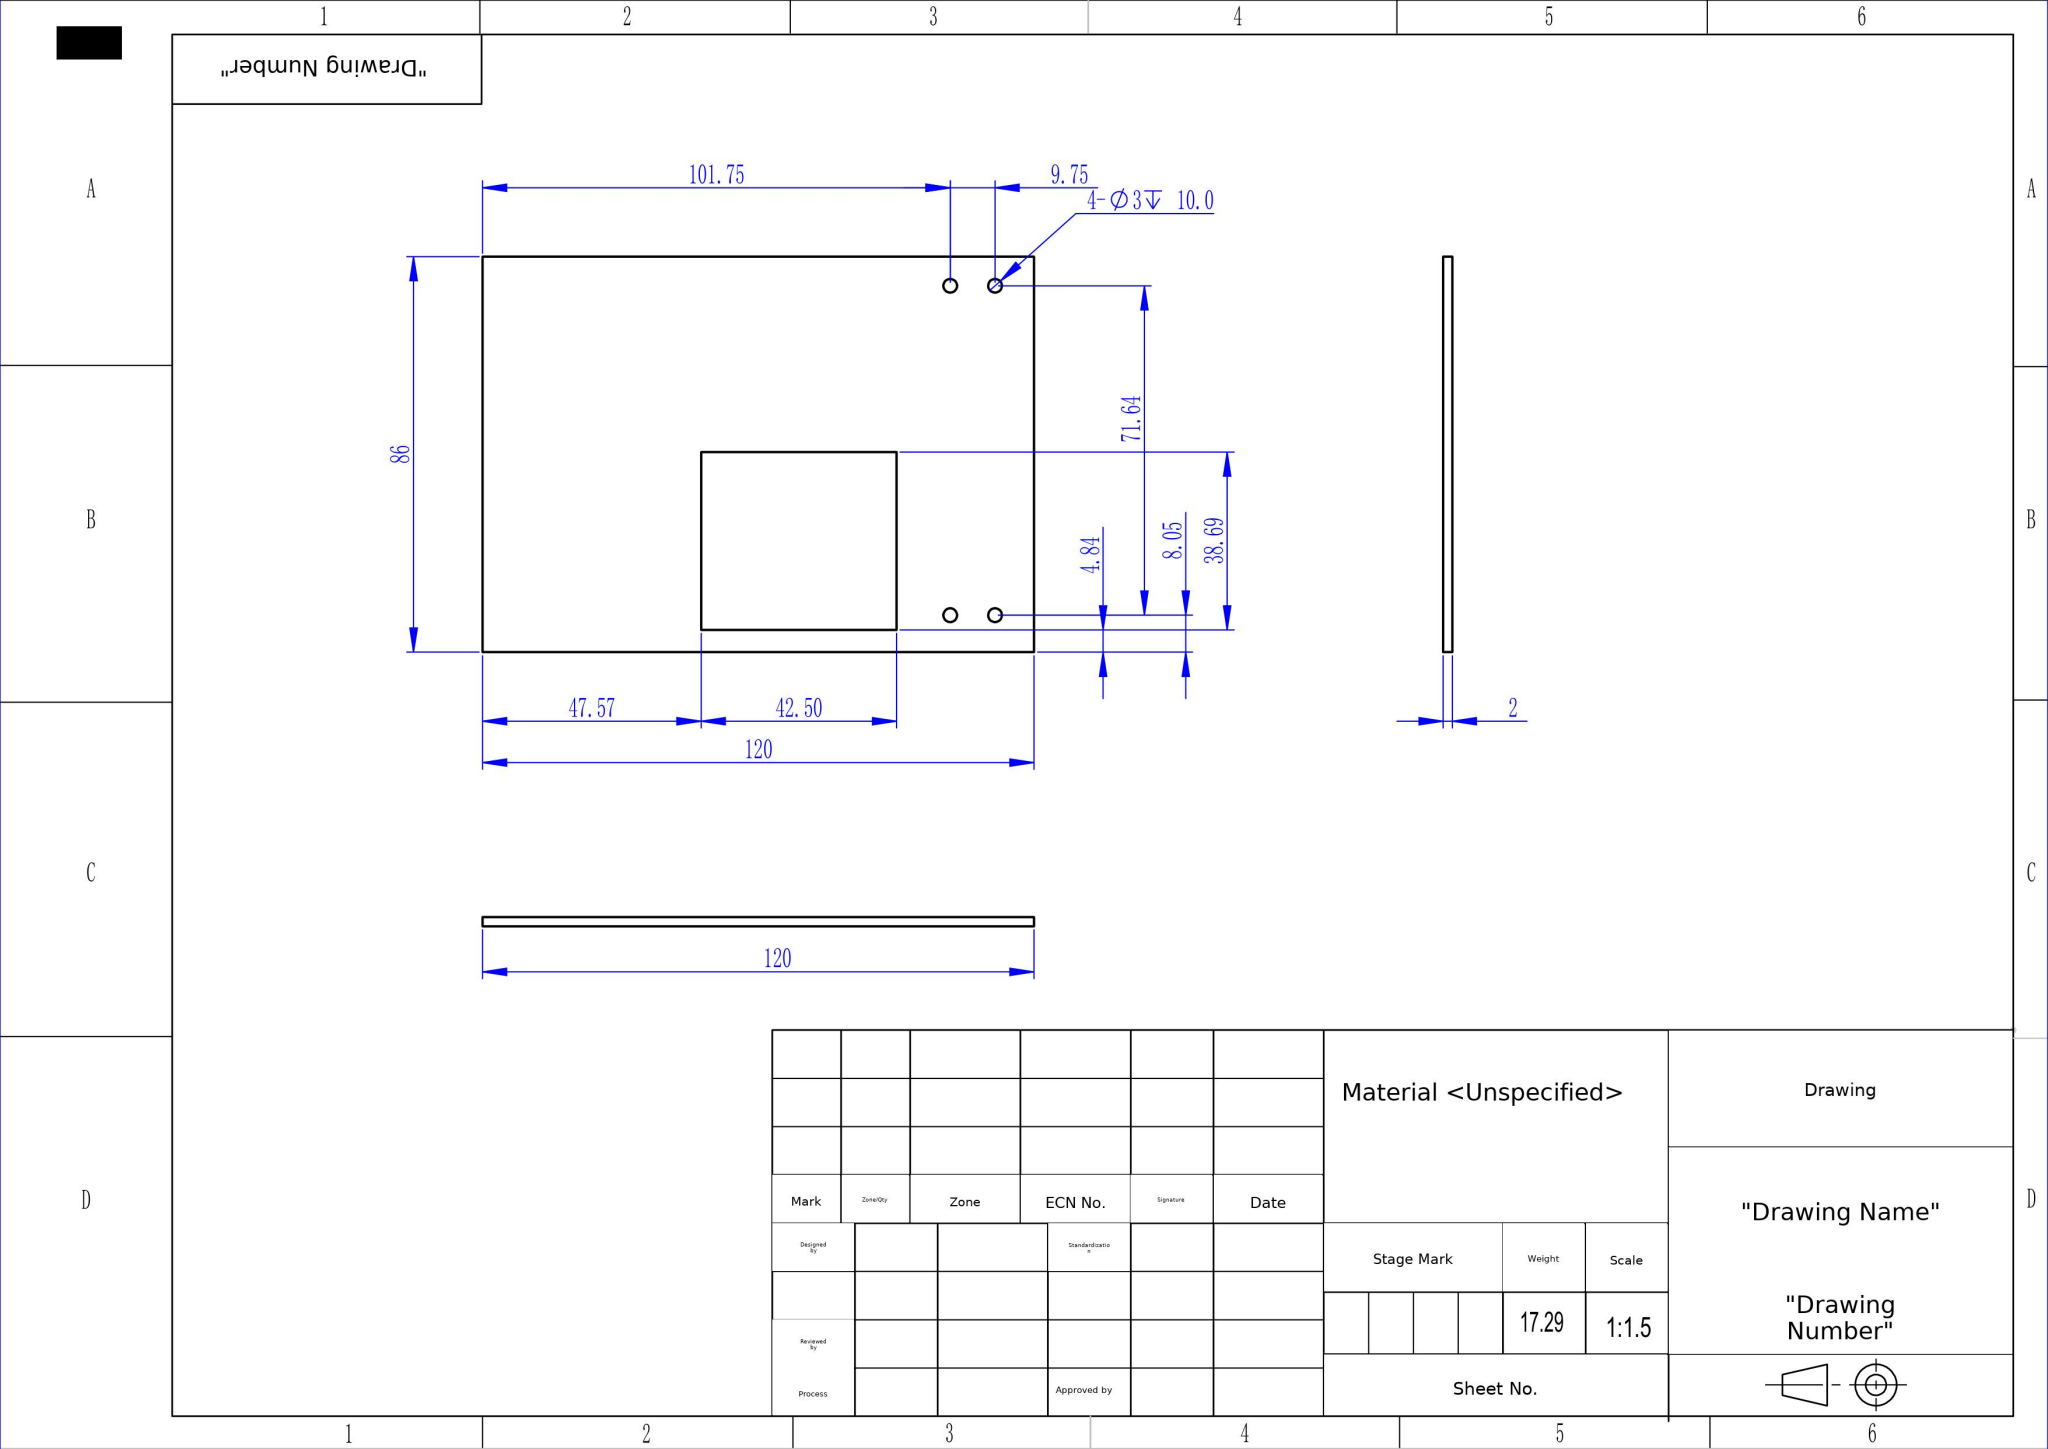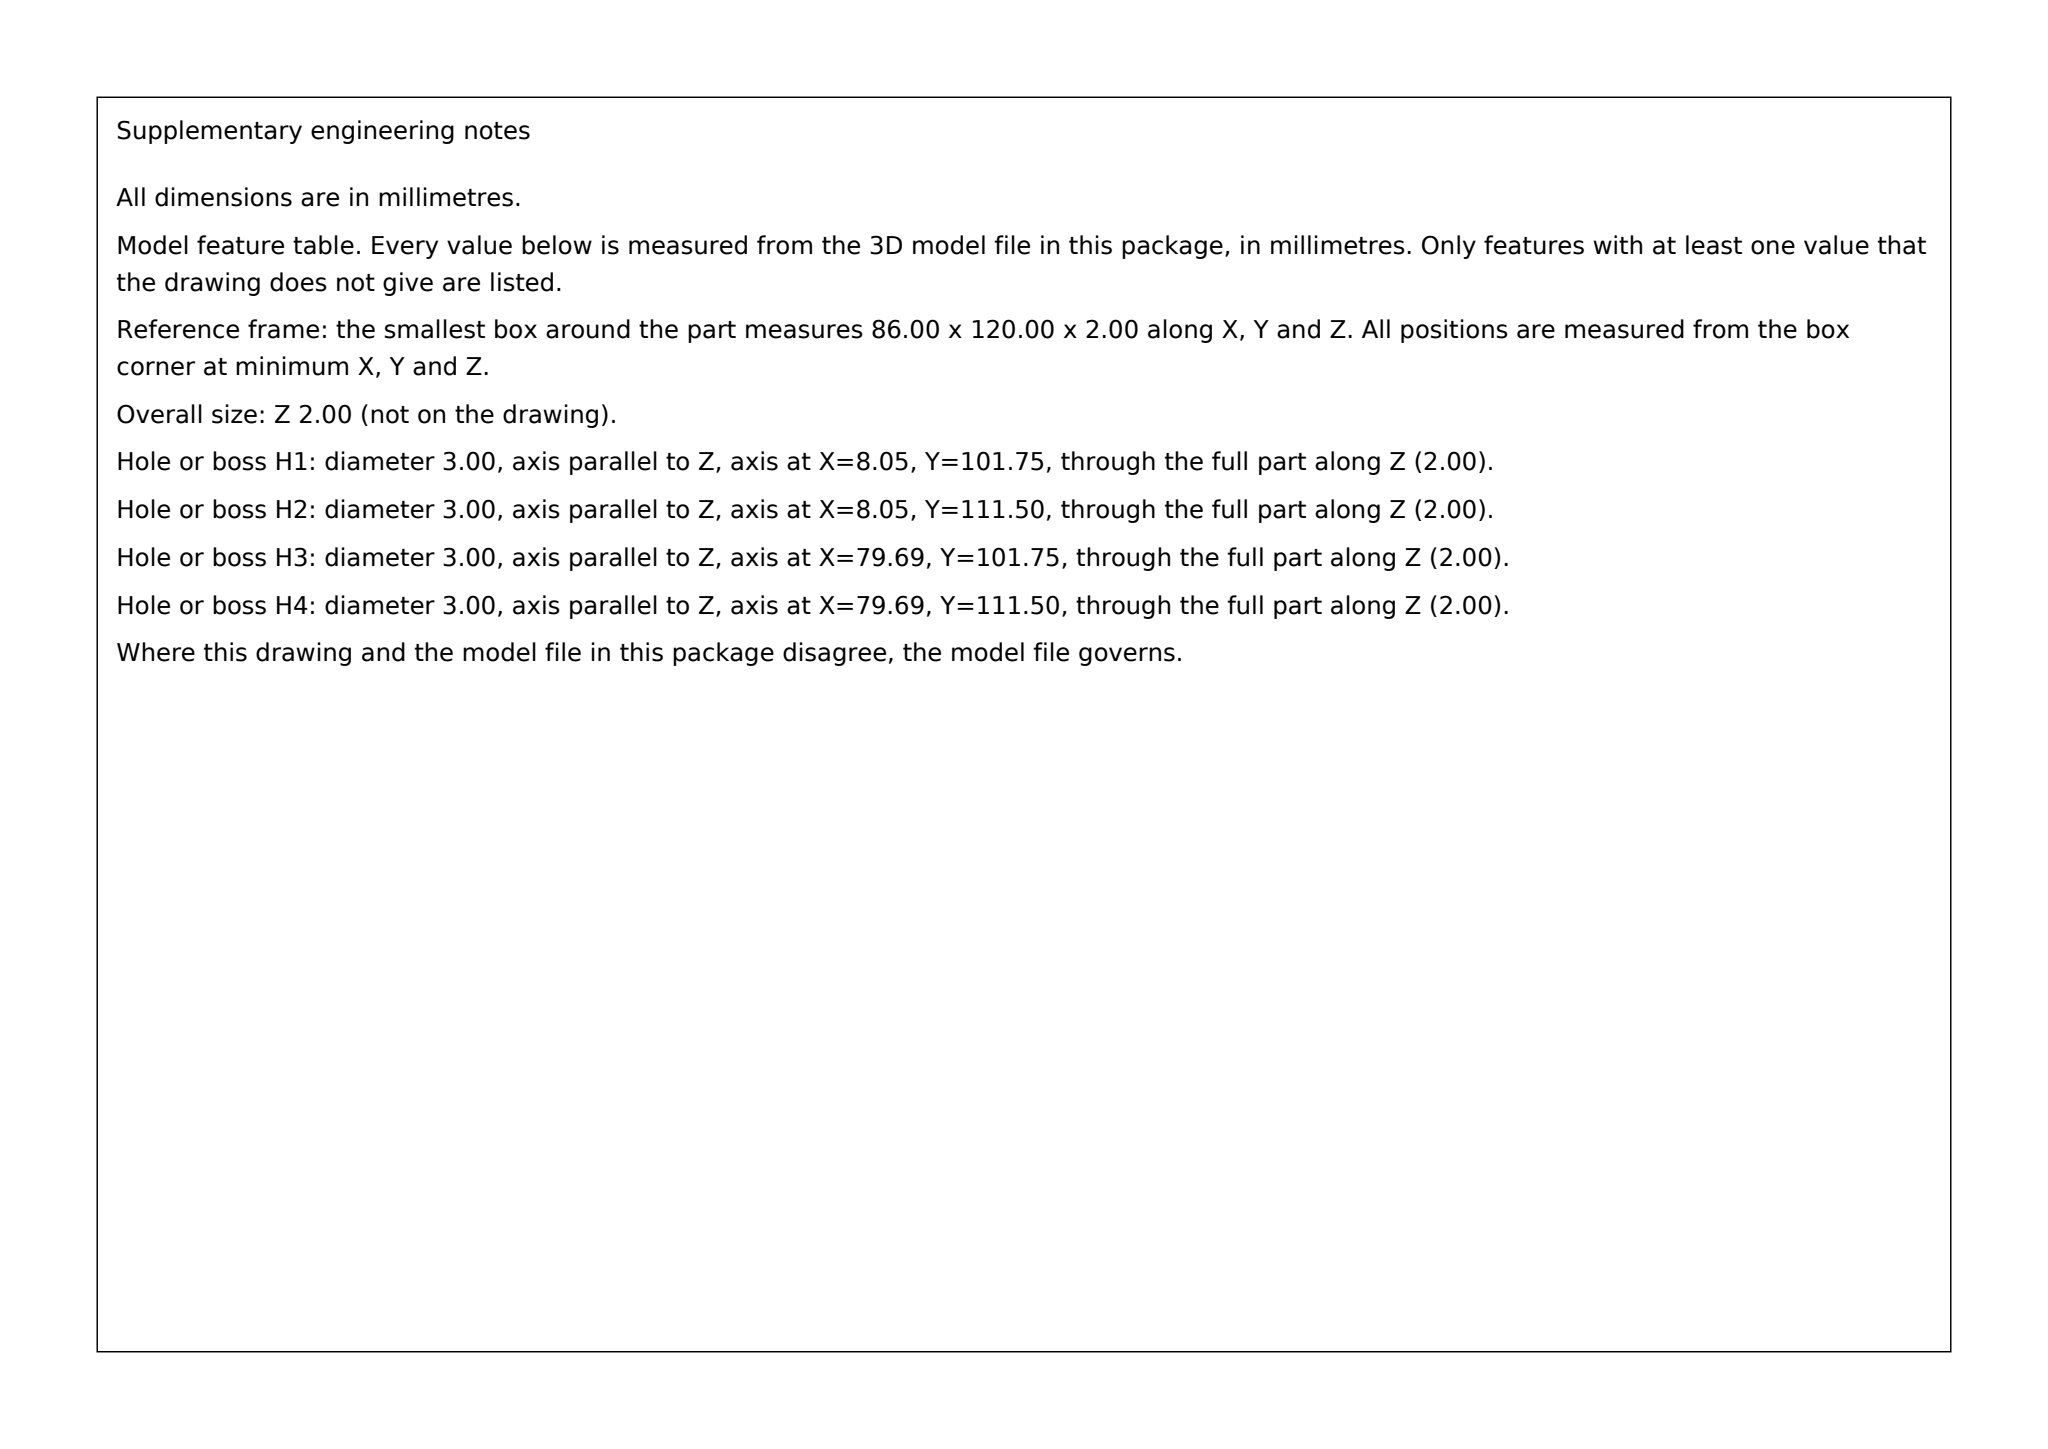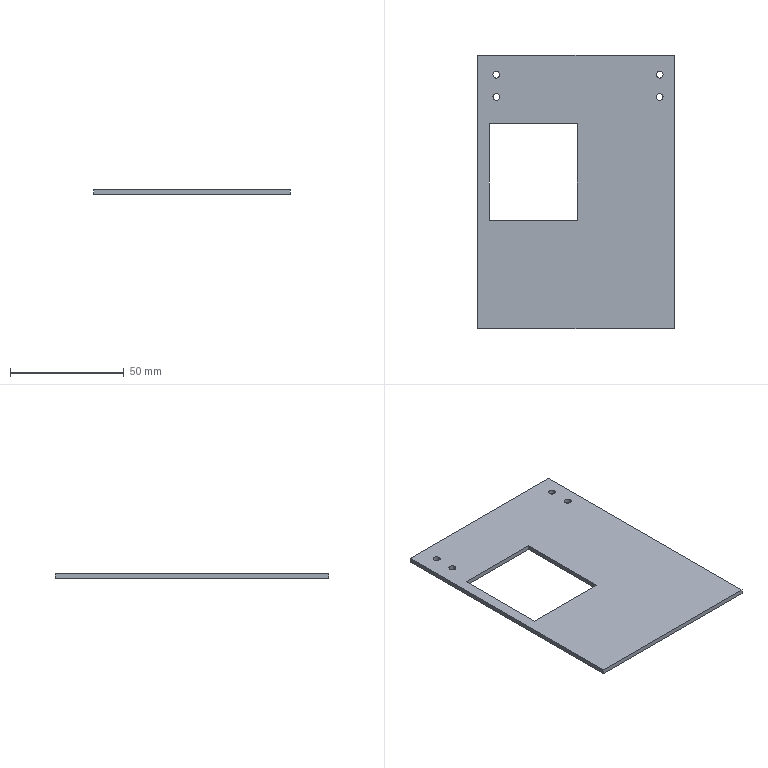Part | SolidWorks | mm | 1 solid | 18 faces | box 86 x 120 x 2 mm | volume 17294 mm3 | plane 10 | cylinder 8 | commonest cylinder face diameters 3 x8
build123d program:
from build123d import *

# Parameters (mm, degrees)
SKETCH1_W           = 86
SKETCH1_H           = 110
BOSS_EXTRUDE1_DEPTH = 2
SKETCH2_R           = 1.5
CUT_EXTRUDE1_DEPTH  = 10
SKETCH3_W           = 38.694
SKETCH3_H           = 42.503
CUT_EXTRUDE2_DEPTH  = 10
SKETCH4_W           = 86
SKETCH4_H           = 10
BOSS_EXTRUDE2_DEPTH = 2


with BuildPart() as part:
    # Sketch1 → Boss-Extrude1 (new body)
    with BuildSketch(Plane.XY):
        Rectangle(SKETCH1_W, SKETCH1_H)
    extrude(amount=BOSS_EXTRUDE1_DEPTH)

    # Sketch2 → Cut-Extrude1 (cut)
    with BuildSketch(Plane(origin=(0, 0, 0), x_dir=(-1, 0, 0), z_dir=(0, 0, -1))):
        with Locations((-36.686, 46.499)):
            Circle(SKETCH2_R)
        with Locations((34.95, 46.499)):
            Circle(SKETCH2_R)
        with Locations((-36.686, 36.747)):
            Circle(SKETCH2_R)
        with Locations((34.95, 36.747)):
            Circle(SKETCH2_R)
    extrude(amount=-CUT_EXTRUDE1_DEPTH, mode=Mode.SUBTRACT)

    # Sketch3 → Cut-Extrude2 (cut)
    with BuildSketch(Plane(origin=(0, 0, 0), x_dir=(-1, 0, 0), z_dir=(0, 0, -1))):
        with Locations((18.817, 3.817)):
            Rectangle(SKETCH3_W, SKETCH3_H)
    extrude(amount=-CUT_EXTRUDE2_DEPTH, mode=Mode.SUBTRACT)

    # Sketch4 → Boss-Extrude2 (add)
    with BuildSketch(Plane.XY.offset(2)):
        with Locations((0, -60)):
            Rectangle(SKETCH4_W, SKETCH4_H)
    extrude(amount=-BOSS_EXTRUDE2_DEPTH)


solid = part.part
STEP:
#1=CARTESIAN_POINT('',(-33.45,46.499,2.));
#2=VERTEX_POINT('',#1);
#3=CARTESIAN_POINT('',(-36.45,46.499,2.));
#4=VERTEX_POINT('',#3);
#5=CARTESIAN_POINT('',(-34.95,46.499,2.));
#6=DIRECTION('',(0.,0.,-1.));
#7=DIRECTION('',(-1.,0.,0.));
#8=AXIS2_PLACEMENT_3D('',#5,#6,#7);
#9=CIRCLE('',#8,1.5);
#10=EDGE_CURVE('',#2,#4,#9,.T.);
#11=ORIENTED_EDGE('',*,*,#10,.F.);
#12=CARTESIAN_POINT('',(-33.45,46.499,0.));
#13=VERTEX_POINT('',#12);
#14=CARTESIAN_POINT('',(-33.45,46.499,10.));
#15=DIRECTION('',(0.,0.,-1.));
#16=VECTOR('',#15,1000.);
#17=LINE('',#14,#16);
#18=EDGE_CURVE('',#2,#13,#17,.T.);
#19=ORIENTED_EDGE('',*,*,#18,.T.);
#20=CARTESIAN_POINT('',(-36.45,46.499,0.));
#21=VERTEX_POINT('',#20);
#22=CARTESIAN_POINT('',(-34.95,46.499,0.));
#23=DIRECTION('',(0.,0.,-1.));
#24=DIRECTION('',(-1.,0.,0.));
#25=AXIS2_PLACEMENT_3D('',#22,#23,#24);
#26=CIRCLE('',#25,1.5);
#27=EDGE_CURVE('',#13,#21,#26,.T.);
#28=ORIENTED_EDGE('',*,*,#27,.T.);
#29=CARTESIAN_POINT('',(-36.45,46.499,10.));
#30=DIRECTION('',(0.,0.,-1.));
#31=VECTOR('',#30,1000.);
#32=LINE('',#29,#31);
#33=EDGE_CURVE('',#4,#21,#32,.T.);
#34=ORIENTED_EDGE('',*,*,#33,.F.);
#35=EDGE_LOOP('',(#11,#19,#28,#34));
#36=FACE_OUTER_BOUND('',#35,.T.);
#37=CARTESIAN_POINT('',(-34.95,46.499,10.));
#38=DIRECTION('',(0.,0.,-1.));
#39=DIRECTION('',(-1.,0.,0.));
#40=AXIS2_PLACEMENT_3D('',#37,#38,#39);
#41=CYLINDRICAL_SURFACE('',#40,1.5);
#42=ADVANCED_FACE('',(#36),#41,.F.);
#43=CARTESIAN_POINT('',(38.186,36.747,2.));
#44=VERTEX_POINT('',#43);
#45=CARTESIAN_POINT('',(35.186,36.747,2.));
#46=VERTEX_POINT('',#45);
#47=CARTESIAN_POINT('',(36.686,36.747,2.));
#48=DIRECTION('',(0.,0.,-1.));
#49=DIRECTION('',(-1.,0.,0.));
#50=AXIS2_PLACEMENT_3D('',#47,#48,#49);
#51=CIRCLE('',#50,1.5);
#52=EDGE_CURVE('',#44,#46,#51,.T.);
#53=ORIENTED_EDGE('',*,*,#52,.F.);
#54=CARTESIAN_POINT('',(38.186,36.747,0.));
#55=VERTEX_POINT('',#54);
#56=CARTESIAN_POINT('',(38.186,36.747,10.));
#57=DIRECTION('',(0.,0.,-1.));
#58=VECTOR('',#57,1000.);
#59=LINE('',#56,#58);
#60=EDGE_CURVE('',#44,#55,#59,.T.);
#61=ORIENTED_EDGE('',*,*,#60,.T.);
#62=CARTESIAN_POINT('',(35.186,36.747,0.));
#63=VERTEX_POINT('',#62);
#64=CARTESIAN_POINT('',(36.686,36.747,0.));
#65=DIRECTION('',(0.,0.,-1.));
#66=DIRECTION('',(-1.,0.,0.));
#67=AXIS2_PLACEMENT_3D('',#64,#65,#66);
#68=CIRCLE('',#67,1.5);
#69=EDGE_CURVE('',#55,#63,#68,.T.);
#70=ORIENTED_EDGE('',*,*,#69,.T.);
#71=CARTESIAN_POINT('',(35.186,36.747,10.));
#72=DIRECTION('',(0.,0.,-1.));
#73=VECTOR('',#72,1000.);
#74=LINE('',#71,#73);
#75=EDGE_CURVE('',#46,#63,#74,.T.);
#76=ORIENTED_EDGE('',*,*,#75,.F.);
#77=EDGE_LOOP('',(#53,#61,#70,#76));
#78=FACE_OUTER_BOUND('',#77,.T.);
#79=CARTESIAN_POINT('',(36.686,36.747,10.));
#80=DIRECTION('',(0.,0.,-1.));
#81=DIRECTION('',(-1.,0.,0.));
#82=AXIS2_PLACEMENT_3D('',#79,#80,#81);
#83=CYLINDRICAL_SURFACE('',#82,1.5);
#84=ADVANCED_FACE('',(#78),#83,.F.);
#85=CARTESIAN_POINT('',(-33.45,36.747,2.));
#86=VERTEX_POINT('',#85);
#87=CARTESIAN_POINT('',(-36.45,36.747,2.));
#88=VERTEX_POINT('',#87);
#89=CARTESIAN_POINT('',(-34.95,36.747,2.));
#90=DIRECTION('',(0.,0.,-1.));
#91=DIRECTION('',(-1.,0.,0.));
#92=AXIS2_PLACEMENT_3D('',#89,#90,#91);
#93=CIRCLE('',#92,1.5);
#94=EDGE_CURVE('',#86,#88,#93,.T.);
#95=ORIENTED_EDGE('',*,*,#94,.F.);
#96=CARTESIAN_POINT('',(-33.45,36.747,0.));
#97=VERTEX_POINT('',#96);
#98=CARTESIAN_POINT('',(-33.45,36.747,10.));
#99=DIRECTION('',(0.,0.,-1.));
#100=VECTOR('',#99,1000.);
#101=LINE('',#98,#100);
#102=EDGE_CURVE('',#86,#97,#101,.T.);
#103=ORIENTED_EDGE('',*,*,#102,.T.);
#104=CARTESIAN_POINT('',(-36.45,36.747,0.));
#105=VERTEX_POINT('',#104);
#106=CARTESIAN_POINT('',(-34.95,36.747,0.));
#107=DIRECTION('',(0.,0.,-1.));
#108=DIRECTION('',(-1.,0.,0.));
#109=AXIS2_PLACEMENT_3D('',#106,#107,#108);
#110=CIRCLE('',#109,1.5);
#111=EDGE_CURVE('',#97,#105,#110,.T.);
#112=ORIENTED_EDGE('',*,*,#111,.T.);
#113=CARTESIAN_POINT('',(-36.45,36.747,10.));
#114=DIRECTION('',(0.,0.,-1.));
#115=VECTOR('',#114,1000.);
#116=LINE('',#113,#115);
#117=EDGE_CURVE('',#88,#105,#116,.T.);
#118=ORIENTED_EDGE('',*,*,#117,.F.);
#119=EDGE_LOOP('',(#95,#103,#112,#118));
#120=FACE_OUTER_BOUND('',#119,.T.);
#121=CARTESIAN_POINT('',(-34.95,36.747,10.));
#122=DIRECTION('',(0.,0.,-1.));
#123=DIRECTION('',(-1.,0.,0.));
#124=AXIS2_PLACEMENT_3D('',#121,#122,#123);
#125=CYLINDRICAL_SURFACE('',#124,1.5);
#126=ADVANCED_FACE('',(#120),#125,.F.);
#127=CARTESIAN_POINT('',(38.186,46.499,2.));
#128=VERTEX_POINT('',#127);
#129=CARTESIAN_POINT('',(35.186,46.499,2.));
#130=VERTEX_POINT('',#129);
#131=CARTESIAN_POINT('',(36.686,46.499,2.));
#132=DIRECTION('',(0.,0.,-1.));
#133=DIRECTION('',(-1.,0.,0.));
#134=AXIS2_PLACEMENT_3D('',#131,#132,#133);
#135=CIRCLE('',#134,1.5);
#136=EDGE_CURVE('',#128,#130,#135,.T.);
#137=ORIENTED_EDGE('',*,*,#136,.F.);
#138=CARTESIAN_POINT('',(38.186,46.499,0.));
#139=VERTEX_POINT('',#138);
#140=CARTESIAN_POINT('',(38.186,46.499,10.));
#141=DIRECTION('',(0.,0.,-1.));
#142=VECTOR('',#141,1000.);
#143=LINE('',#140,#142);
#144=EDGE_CURVE('',#128,#139,#143,.T.);
#145=ORIENTED_EDGE('',*,*,#144,.T.);
#146=CARTESIAN_POINT('',(35.186,46.499,0.));
#147=VERTEX_POINT('',#146);
#148=CARTESIAN_POINT('',(36.686,46.499,0.));
#149=DIRECTION('',(0.,0.,-1.));
#150=DIRECTION('',(-1.,0.,0.));
#151=AXIS2_PLACEMENT_3D('',#148,#149,#150);
#152=CIRCLE('',#151,1.5);
#153=EDGE_CURVE('',#139,#147,#152,.T.);
#154=ORIENTED_EDGE('',*,*,#153,.T.);
#155=CARTESIAN_POINT('',(35.186,46.499,10.));
#156=DIRECTION('',(0.,0.,-1.));
#157=VECTOR('',#156,1000.);
#158=LINE('',#155,#157);
#159=EDGE_CURVE('',#130,#147,#158,.T.);
#160=ORIENTED_EDGE('',*,*,#159,.F.);
#161=EDGE_LOOP('',(#137,#145,#154,#160));
#162=FACE_OUTER_BOUND('',#161,.T.);
#163=CARTESIAN_POINT('',(36.686,46.499,10.));
#164=DIRECTION('',(0.,0.,-1.));
#165=DIRECTION('',(-1.,0.,0.));
#166=AXIS2_PLACEMENT_3D('',#163,#164,#165);
#167=CYLINDRICAL_SURFACE('',#166,1.5);
#168=ADVANCED_FACE('',(#162),#167,.F.);
#169=CARTESIAN_POINT('',(43.,-65.,0.));
#170=VERTEX_POINT('',#169);
#171=CARTESIAN_POINT('',(43.,55.,0.));
#172=VERTEX_POINT('',#171);
#173=CARTESIAN_POINT('',(43.,-55.,0.));
#174=DIRECTION('',(0.,1.,0.));
#175=VECTOR('',#174,1000.);
#176=LINE('',#173,#175);
#177=EDGE_CURVE('',#170,#172,#176,.T.);
#178=ORIENTED_EDGE('',*,*,#177,.T.);
#179=CARTESIAN_POINT('',(43.,55.,2.));
#180=VERTEX_POINT('',#179);
#181=CARTESIAN_POINT('',(43.,55.,2.));
#182=DIRECTION('',(0.,0.,-1.));
#183=VECTOR('',#182,1000.);
#184=LINE('',#181,#183);
#185=EDGE_CURVE('',#180,#172,#184,.T.);
#186=ORIENTED_EDGE('',*,*,#185,.F.);
#187=CARTESIAN_POINT('',(43.,-65.,2.));
#188=VERTEX_POINT('',#187);
#189=CARTESIAN_POINT('',(43.,-55.,2.));
#190=DIRECTION('',(0.,1.,0.));
#191=VECTOR('',#190,1000.);
#192=LINE('',#189,#191);
#193=EDGE_CURVE('',#188,#180,#192,.T.);
#194=ORIENTED_EDGE('',*,*,#193,.F.);
#195=CARTESIAN_POINT('',(43.,-65.,0.));
#196=DIRECTION('',(0.,0.,1.));
#197=VECTOR('',#196,1000.);
#198=LINE('',#195,#197);
#199=EDGE_CURVE('',#170,#188,#198,.T.);
#200=ORIENTED_EDGE('',*,*,#199,.F.);
#201=EDGE_LOOP('',(#178,#186,#194,#200));
#202=FACE_OUTER_BOUND('',#201,.T.);
#203=CARTESIAN_POINT('',(43.,-55.,2.));
#204=DIRECTION('',(-1.,0.,0.));
#205=DIRECTION('',(0.,0.,1.));
#206=AXIS2_PLACEMENT_3D('',#203,#204,#205);
#207=PLANE('',#206);
#208=ADVANCED_FACE('',(#202),#207,.F.);
#209=CARTESIAN_POINT('',(-43.,55.,0.));
#210=VERTEX_POINT('',#209);
#211=CARTESIAN_POINT('',(-43.,55.,0.));
#212=DIRECTION('',(-1.,0.,0.));
#213=VECTOR('',#212,1000.);
#214=LINE('',#211,#213);
#215=EDGE_CURVE('',#172,#210,#214,.T.);
#216=ORIENTED_EDGE('',*,*,#215,.T.);
#217=CARTESIAN_POINT('',(-43.,55.,2.));
#218=VERTEX_POINT('',#217);
#219=CARTESIAN_POINT('',(-43.,55.,2.));
#220=DIRECTION('',(0.,0.,-1.));
#221=VECTOR('',#220,1000.);
#222=LINE('',#219,#221);
#223=EDGE_CURVE('',#218,#210,#222,.T.);
#224=ORIENTED_EDGE('',*,*,#223,.F.);
#225=CARTESIAN_POINT('',(-43.,55.,2.));
#226=DIRECTION('',(-1.,0.,0.));
#227=VECTOR('',#226,1000.);
#228=LINE('',#225,#227);
#229=EDGE_CURVE('',#180,#218,#228,.T.);
#230=ORIENTED_EDGE('',*,*,#229,.F.);
#231=ORIENTED_EDGE('',*,*,#185,.T.);
#232=EDGE_LOOP('',(#216,#224,#230,#231));
#233=FACE_OUTER_BOUND('',#232,.T.);
#234=CARTESIAN_POINT('',(-43.,55.,2.));
#235=DIRECTION('',(0.,-1.,0.));
#236=DIRECTION('',(0.,0.,-1.));
#237=AXIS2_PLACEMENT_3D('',#234,#235,#236);
#238=PLANE('',#237);
#239=ADVANCED_FACE('',(#233),#238,.F.);
#240=CARTESIAN_POINT('',(-43.,-65.,0.));
#241=VERTEX_POINT('',#240);
#242=CARTESIAN_POINT('',(-43.,-55.,0.));
#243=DIRECTION('',(0.,-1.,0.));
#244=VECTOR('',#243,1000.);
#245=LINE('',#242,#244);
#246=EDGE_CURVE('',#210,#241,#245,.T.);
#247=ORIENTED_EDGE('',*,*,#246,.T.);
#248=CARTESIAN_POINT('',(-43.,-65.,2.));
#249=VERTEX_POINT('',#248);
#250=CARTESIAN_POINT('',(-43.,-65.,0.));
#251=DIRECTION('',(0.,0.,1.));
#252=VECTOR('',#251,1000.);
#253=LINE('',#250,#252);
#254=EDGE_CURVE('',#241,#249,#253,.T.);
#255=ORIENTED_EDGE('',*,*,#254,.T.);
#256=CARTESIAN_POINT('',(-43.,-55.,2.));
#257=DIRECTION('',(0.,-1.,0.));
#258=VECTOR('',#257,1000.);
#259=LINE('',#256,#258);
#260=EDGE_CURVE('',#218,#249,#259,.T.);
#261=ORIENTED_EDGE('',*,*,#260,.F.);
#262=ORIENTED_EDGE('',*,*,#223,.T.);
#263=EDGE_LOOP('',(#247,#255,#261,#262));
#264=FACE_OUTER_BOUND('',#263,.T.);
#265=CARTESIAN_POINT('',(-43.,-55.,2.));
#266=DIRECTION('',(1.,0.,0.));
#267=DIRECTION('',(0.,0.,-1.));
#268=AXIS2_PLACEMENT_3D('',#265,#266,#267);
#269=PLANE('',#268);
#270=ADVANCED_FACE('',(#264),#269,.F.);
#271=CARTESIAN_POINT('',(0.5299,-17.435,2.));
#272=VERTEX_POINT('',#271);
#273=CARTESIAN_POINT('',(-38.164,-17.435,2.));
#274=VERTEX_POINT('',#273);
#275=CARTESIAN_POINT('',(0.,-17.435,2.));
#276=DIRECTION('',(-1.,0.,0.));
#277=VECTOR('',#276,1000.);
#278=LINE('',#275,#277);
#279=EDGE_CURVE('',#272,#274,#278,.T.);
#280=ORIENTED_EDGE('',*,*,#279,.T.);
#281=CARTESIAN_POINT('',(-38.164,25.068,2.));
#282=VERTEX_POINT('',#281);
#283=CARTESIAN_POINT('',(-38.164,0.,2.));
#284=DIRECTION('',(0.,1.,0.));
#285=VECTOR('',#284,1000.);
#286=LINE('',#283,#285);
#287=EDGE_CURVE('',#274,#282,#286,.T.);
#288=ORIENTED_EDGE('',*,*,#287,.T.);
#289=CARTESIAN_POINT('',(0.5299,25.068,2.));
#290=VERTEX_POINT('',#289);
#291=CARTESIAN_POINT('',(0.,25.068,2.));
#292=DIRECTION('',(1.,0.,0.));
#293=VECTOR('',#292,1000.);
#294=LINE('',#291,#293);
#295=EDGE_CURVE('',#282,#290,#294,.T.);
#296=ORIENTED_EDGE('',*,*,#295,.T.);
#297=CARTESIAN_POINT('',(0.5299,0.,2.));
#298=DIRECTION('',(0.,-1.,0.));
#299=VECTOR('',#298,1000.);
#300=LINE('',#297,#299);
#301=EDGE_CURVE('',#290,#272,#300,.T.);
#302=ORIENTED_EDGE('',*,*,#301,.T.);
#303=EDGE_LOOP('',(#280,#288,#296,#302));
#304=FACE_BOUND('',#303,.T.);
#305=CARTESIAN_POINT('',(-34.95,46.499,2.));
#306=DIRECTION('',(0.,0.,-1.));
#307=DIRECTION('',(-1.,0.,0.));
#308=AXIS2_PLACEMENT_3D('',#305,#306,#307);
#309=CIRCLE('',#308,1.5);
#310=EDGE_CURVE('',#4,#2,#309,.T.);
#311=ORIENTED_EDGE('',*,*,#310,.T.);
#312=ORIENTED_EDGE('',*,*,#10,.T.);
#313=EDGE_LOOP('',(#311,#312));
#314=FACE_BOUND('',#313,.T.);
#315=CARTESIAN_POINT('',(36.686,36.747,2.));
#316=DIRECTION('',(0.,0.,-1.));
#317=DIRECTION('',(-1.,0.,0.));
#318=AXIS2_PLACEMENT_3D('',#315,#316,#317);
#319=CIRCLE('',#318,1.5);
#320=EDGE_CURVE('',#46,#44,#319,.T.);
#321=ORIENTED_EDGE('',*,*,#320,.T.);
#322=ORIENTED_EDGE('',*,*,#52,.T.);
#323=EDGE_LOOP('',(#321,#322));
#324=FACE_BOUND('',#323,.T.);
#325=CARTESIAN_POINT('',(-34.95,36.747,2.));
#326=DIRECTION('',(0.,0.,-1.));
#327=DIRECTION('',(-1.,0.,0.));
#328=AXIS2_PLACEMENT_3D('',#325,#326,#327);
#329=CIRCLE('',#328,1.5);
#330=EDGE_CURVE('',#88,#86,#329,.T.);
#331=ORIENTED_EDGE('',*,*,#330,.T.);
#332=ORIENTED_EDGE('',*,*,#94,.T.);
#333=EDGE_LOOP('',(#331,#332));
#334=FACE_BOUND('',#333,.T.);
#335=CARTESIAN_POINT('',(36.686,46.499,2.));
#336=DIRECTION('',(0.,0.,-1.));
#337=DIRECTION('',(-1.,0.,0.));
#338=AXIS2_PLACEMENT_3D('',#335,#336,#337);
#339=CIRCLE('',#338,1.5);
#340=EDGE_CURVE('',#130,#128,#339,.T.);
#341=ORIENTED_EDGE('',*,*,#340,.T.);
#342=ORIENTED_EDGE('',*,*,#136,.T.);
#343=EDGE_LOOP('',(#341,#342));
#344=FACE_BOUND('',#343,.T.);
#345=ORIENTED_EDGE('',*,*,#193,.T.);
#346=ORIENTED_EDGE('',*,*,#229,.T.);
#347=ORIENTED_EDGE('',*,*,#260,.T.);
#348=CARTESIAN_POINT('',(-43.,-65.,2.));
#349=DIRECTION('',(1.,0.,0.));
#350=VECTOR('',#349,1000.);
#351=LINE('',#348,#350);
#352=EDGE_CURVE('',#249,#188,#351,.T.);
#353=ORIENTED_EDGE('',*,*,#352,.T.);
#354=EDGE_LOOP('',(#345,#346,#347,#353));
#355=FACE_OUTER_BOUND('',#354,.T.);
#356=CARTESIAN_POINT('',(0.,0.,2.));
#357=DIRECTION('',(0.,0.,-1.));
#358=DIRECTION('',(-1.,0.,0.));
#359=AXIS2_PLACEMENT_3D('',#356,#357,#358);
#360=PLANE('',#359);
#361=ADVANCED_FACE('',(#304,#314,#324,#334,#344,#355),#360,.F.);
#362=CARTESIAN_POINT('',(-38.164,-17.435,0.));
#363=VERTEX_POINT('',#362);
#364=CARTESIAN_POINT('',(-38.164,25.068,0.));
#365=VERTEX_POINT('',#364);
#366=CARTESIAN_POINT('',(-38.164,-17.435,0.));
#367=DIRECTION('',(0.,1.,0.));
#368=VECTOR('',#367,1000.);
#369=LINE('',#366,#368);
#370=EDGE_CURVE('',#363,#365,#369,.T.);
#371=ORIENTED_EDGE('',*,*,#370,.F.);
#372=CARTESIAN_POINT('',(0.5299,-17.435,0.));
#373=VERTEX_POINT('',#372);
#374=CARTESIAN_POINT('',(0.5299,-17.435,0.));
#375=DIRECTION('',(-1.,0.,0.));
#376=VECTOR('',#375,1000.);
#377=LINE('',#374,#376);
#378=EDGE_CURVE('',#373,#363,#377,.T.);
#379=ORIENTED_EDGE('',*,*,#378,.F.);
#380=CARTESIAN_POINT('',(0.5299,25.068,0.));
#381=VERTEX_POINT('',#380);
#382=CARTESIAN_POINT('',(0.5299,-17.435,0.));
#383=DIRECTION('',(0.,-1.,0.));
#384=VECTOR('',#383,1000.);
#385=LINE('',#382,#384);
#386=EDGE_CURVE('',#381,#373,#385,.T.);
#387=ORIENTED_EDGE('',*,*,#386,.F.);
#388=CARTESIAN_POINT('',(0.5299,25.068,0.));
#389=DIRECTION('',(1.,0.,0.));
#390=VECTOR('',#389,1000.);
#391=LINE('',#388,#390);
#392=EDGE_CURVE('',#365,#381,#391,.T.);
#393=ORIENTED_EDGE('',*,*,#392,.F.);
#394=EDGE_LOOP('',(#371,#379,#387,#393));
#395=FACE_BOUND('',#394,.T.);
#396=CARTESIAN_POINT('',(-34.95,46.499,0.));
#397=DIRECTION('',(0.,0.,-1.));
#398=DIRECTION('',(-1.,0.,0.));
#399=AXIS2_PLACEMENT_3D('',#396,#397,#398);
#400=CIRCLE('',#399,1.5);
#401=EDGE_CURVE('',#21,#13,#400,.T.);
#402=ORIENTED_EDGE('',*,*,#401,.F.);
#403=ORIENTED_EDGE('',*,*,#27,.F.);
#404=EDGE_LOOP('',(#402,#403));
#405=FACE_BOUND('',#404,.T.);
#406=CARTESIAN_POINT('',(36.686,36.747,0.));
#407=DIRECTION('',(0.,0.,-1.));
#408=DIRECTION('',(-1.,0.,0.));
#409=AXIS2_PLACEMENT_3D('',#406,#407,#408);
#410=CIRCLE('',#409,1.5);
#411=EDGE_CURVE('',#63,#55,#410,.T.);
#412=ORIENTED_EDGE('',*,*,#411,.F.);
#413=ORIENTED_EDGE('',*,*,#69,.F.);
#414=EDGE_LOOP('',(#412,#413));
#415=FACE_BOUND('',#414,.T.);
#416=CARTESIAN_POINT('',(-34.95,36.747,0.));
#417=DIRECTION('',(0.,0.,-1.));
#418=DIRECTION('',(-1.,0.,0.));
#419=AXIS2_PLACEMENT_3D('',#416,#417,#418);
#420=CIRCLE('',#419,1.5);
#421=EDGE_CURVE('',#105,#97,#420,.T.);
#422=ORIENTED_EDGE('',*,*,#421,.F.);
#423=ORIENTED_EDGE('',*,*,#111,.F.);
#424=EDGE_LOOP('',(#422,#423));
#425=FACE_BOUND('',#424,.T.);
#426=CARTESIAN_POINT('',(36.686,46.499,0.));
#427=DIRECTION('',(0.,0.,-1.));
#428=DIRECTION('',(-1.,0.,0.));
#429=AXIS2_PLACEMENT_3D('',#426,#427,#428);
#430=CIRCLE('',#429,1.5);
#431=EDGE_CURVE('',#147,#139,#430,.T.);
#432=ORIENTED_EDGE('',*,*,#431,.F.);
#433=ORIENTED_EDGE('',*,*,#153,.F.);
#434=EDGE_LOOP('',(#432,#433));
#435=FACE_BOUND('',#434,.T.);
#436=ORIENTED_EDGE('',*,*,#177,.F.);
#437=CARTESIAN_POINT('',(-43.,-65.,0.));
#438=DIRECTION('',(1.,0.,0.));
#439=VECTOR('',#438,1000.);
#440=LINE('',#437,#439);
#441=EDGE_CURVE('',#241,#170,#440,.T.);
#442=ORIENTED_EDGE('',*,*,#441,.F.);
#443=ORIENTED_EDGE('',*,*,#246,.F.);
#444=ORIENTED_EDGE('',*,*,#215,.F.);
#445=EDGE_LOOP('',(#436,#442,#443,#444));
#446=FACE_OUTER_BOUND('',#445,.T.);
#447=CARTESIAN_POINT('',(0.,0.,0.));
#448=DIRECTION('',(0.,0.,-1.));
#449=DIRECTION('',(-1.,0.,0.));
#450=AXIS2_PLACEMENT_3D('',#447,#448,#449);
#451=PLANE('',#450);
#452=ADVANCED_FACE('',(#395,#405,#415,#425,#435,#446),#451,.T.);
#453=ORIENTED_EDGE('',*,*,#144,.F.);
#454=ORIENTED_EDGE('',*,*,#340,.F.);
#455=ORIENTED_EDGE('',*,*,#159,.T.);
#456=ORIENTED_EDGE('',*,*,#431,.T.);
#457=EDGE_LOOP('',(#453,#454,#455,#456));
#458=FACE_OUTER_BOUND('',#457,.T.);
#459=CARTESIAN_POINT('',(36.686,46.499,10.));
#460=DIRECTION('',(0.,0.,-1.));
#461=DIRECTION('',(-1.,0.,0.));
#462=AXIS2_PLACEMENT_3D('',#459,#460,#461);
#463=CYLINDRICAL_SURFACE('',#462,1.5);
#464=ADVANCED_FACE('',(#458),#463,.F.);
#465=ORIENTED_EDGE('',*,*,#102,.F.);
#466=ORIENTED_EDGE('',*,*,#330,.F.);
#467=ORIENTED_EDGE('',*,*,#117,.T.);
#468=ORIENTED_EDGE('',*,*,#421,.T.);
#469=EDGE_LOOP('',(#465,#466,#467,#468));
#470=FACE_OUTER_BOUND('',#469,.T.);
#471=CARTESIAN_POINT('',(-34.95,36.747,10.));
#472=DIRECTION('',(0.,0.,-1.));
#473=DIRECTION('',(-1.,0.,0.));
#474=AXIS2_PLACEMENT_3D('',#471,#472,#473);
#475=CYLINDRICAL_SURFACE('',#474,1.5);
#476=ADVANCED_FACE('',(#470),#475,.F.);
#477=ORIENTED_EDGE('',*,*,#60,.F.);
#478=ORIENTED_EDGE('',*,*,#320,.F.);
#479=ORIENTED_EDGE('',*,*,#75,.T.);
#480=ORIENTED_EDGE('',*,*,#411,.T.);
#481=EDGE_LOOP('',(#477,#478,#479,#480));
#482=FACE_OUTER_BOUND('',#481,.T.);
#483=CARTESIAN_POINT('',(36.686,36.747,10.));
#484=DIRECTION('',(0.,0.,-1.));
#485=DIRECTION('',(-1.,0.,0.));
#486=AXIS2_PLACEMENT_3D('',#483,#484,#485);
#487=CYLINDRICAL_SURFACE('',#486,1.5);
#488=ADVANCED_FACE('',(#482),#487,.F.);
#489=ORIENTED_EDGE('',*,*,#18,.F.);
#490=ORIENTED_EDGE('',*,*,#310,.F.);
#491=ORIENTED_EDGE('',*,*,#33,.T.);
#492=ORIENTED_EDGE('',*,*,#401,.T.);
#493=EDGE_LOOP('',(#489,#490,#491,#492));
#494=FACE_OUTER_BOUND('',#493,.T.);
#495=CARTESIAN_POINT('',(-34.95,46.499,10.));
#496=DIRECTION('',(0.,0.,-1.));
#497=DIRECTION('',(-1.,0.,0.));
#498=AXIS2_PLACEMENT_3D('',#495,#496,#497);
#499=CYLINDRICAL_SURFACE('',#498,1.5);
#500=ADVANCED_FACE('',(#494),#499,.F.);
#501=CARTESIAN_POINT('',(-38.164,-17.435,10.));
#502=DIRECTION('',(0.,0.,-1.));
#503=VECTOR('',#502,1000.);
#504=LINE('',#501,#503);
#505=EDGE_CURVE('',#274,#363,#504,.T.);
#506=ORIENTED_EDGE('',*,*,#505,.T.);
#507=ORIENTED_EDGE('',*,*,#370,.T.);
#508=CARTESIAN_POINT('',(-38.164,25.068,10.));
#509=DIRECTION('',(0.,0.,-1.));
#510=VECTOR('',#509,1000.);
#511=LINE('',#508,#510);
#512=EDGE_CURVE('',#282,#365,#511,.T.);
#513=ORIENTED_EDGE('',*,*,#512,.F.);
#514=ORIENTED_EDGE('',*,*,#287,.F.);
#515=EDGE_LOOP('',(#506,#507,#513,#514));
#516=FACE_OUTER_BOUND('',#515,.T.);
#517=CARTESIAN_POINT('',(-38.164,-17.435,10.));
#518=DIRECTION('',(-1.,0.,0.));
#519=DIRECTION('',(0.,0.,1.));
#520=AXIS2_PLACEMENT_3D('',#517,#518,#519);
#521=PLANE('',#520);
#522=ADVANCED_FACE('',(#516),#521,.F.);
#523=CARTESIAN_POINT('',(0.5299,-17.435,10.));
#524=DIRECTION('',(0.,0.,-1.));
#525=VECTOR('',#524,1000.);
#526=LINE('',#523,#525);
#527=EDGE_CURVE('',#272,#373,#526,.T.);
#528=ORIENTED_EDGE('',*,*,#527,.T.);
#529=ORIENTED_EDGE('',*,*,#378,.T.);
#530=ORIENTED_EDGE('',*,*,#505,.F.);
#531=ORIENTED_EDGE('',*,*,#279,.F.);
#532=EDGE_LOOP('',(#528,#529,#530,#531));
#533=FACE_OUTER_BOUND('',#532,.T.);
#534=CARTESIAN_POINT('',(0.5299,-17.435,10.));
#535=DIRECTION('',(0.,-1.,0.));
#536=DIRECTION('',(0.,0.,-1.));
#537=AXIS2_PLACEMENT_3D('',#534,#535,#536);
#538=PLANE('',#537);
#539=ADVANCED_FACE('',(#533),#538,.F.);
#540=CARTESIAN_POINT('',(0.5299,25.068,10.));
#541=DIRECTION('',(0.,0.,-1.));
#542=VECTOR('',#541,1000.);
#543=LINE('',#540,#542);
#544=EDGE_CURVE('',#290,#381,#543,.T.);
#545=ORIENTED_EDGE('',*,*,#544,.T.);
#546=ORIENTED_EDGE('',*,*,#386,.T.);
#547=ORIENTED_EDGE('',*,*,#527,.F.);
#548=ORIENTED_EDGE('',*,*,#301,.F.);
#549=EDGE_LOOP('',(#545,#546,#547,#548));
#550=FACE_OUTER_BOUND('',#549,.T.);
#551=CARTESIAN_POINT('',(0.5299,-17.435,10.));
#552=DIRECTION('',(1.,0.,0.));
#553=DIRECTION('',(0.,0.,-1.));
#554=AXIS2_PLACEMENT_3D('',#551,#552,#553);
#555=PLANE('',#554);
#556=ADVANCED_FACE('',(#550),#555,.F.);
#557=ORIENTED_EDGE('',*,*,#512,.T.);
#558=ORIENTED_EDGE('',*,*,#392,.T.);
#559=ORIENTED_EDGE('',*,*,#544,.F.);
#560=ORIENTED_EDGE('',*,*,#295,.F.);
#561=EDGE_LOOP('',(#557,#558,#559,#560));
#562=FACE_OUTER_BOUND('',#561,.T.);
#563=CARTESIAN_POINT('',(0.5299,25.068,10.));
#564=DIRECTION('',(0.,1.,0.));
#565=DIRECTION('',(0.,0.,1.));
#566=AXIS2_PLACEMENT_3D('',#563,#564,#565);
#567=PLANE('',#566);
#568=ADVANCED_FACE('',(#562),#567,.F.);
#569=ORIENTED_EDGE('',*,*,#352,.F.);
#570=ORIENTED_EDGE('',*,*,#254,.F.);
#571=ORIENTED_EDGE('',*,*,#441,.T.);
#572=ORIENTED_EDGE('',*,*,#199,.T.);
#573=EDGE_LOOP('',(#569,#570,#571,#572));
#574=FACE_OUTER_BOUND('',#573,.T.);
#575=CARTESIAN_POINT('',(-43.,-65.,0.));
#576=DIRECTION('',(0.,-1.,0.));
#577=DIRECTION('',(0.,0.,-1.));
#578=AXIS2_PLACEMENT_3D('',#575,#576,#577);
#579=PLANE('',#578);
#580=ADVANCED_FACE('',(#574),#579,.T.);
#581=CLOSED_SHELL('',(#42,#84,#126,#168,#208,#239,#270,#361,#452,#464,#476,#488,#500,#522,#539,#556,#568,#580));
#582=MANIFOLD_SOLID_BREP('',#581);
#583=CARTESIAN_POINT('',(0.,0.,0.));
#584=DIRECTION('',(0.,0.,1.));
#585=DIRECTION('',(1.,0.,0.));
#586=AXIS2_PLACEMENT_3D('',#583,#584,#585);
#587=(LENGTH_UNIT()NAMED_UNIT(*)SI_UNIT(.MILLI.,.METRE.));
#588=UNCERTAINTY_MEASURE_WITH_UNIT(LENGTH_MEASURE(0.00001),#587,'','');
#589=(NAMED_UNIT(*)PLANE_ANGLE_UNIT()SI_UNIT($,.RADIAN.));
#590=(NAMED_UNIT(*)SI_UNIT($,.STERADIAN.)SOLID_ANGLE_UNIT());
#591=(GEOMETRIC_REPRESENTATION_CONTEXT(3)GLOBAL_UNCERTAINTY_ASSIGNED_CONTEXT((#588))GLOBAL_UNIT_ASSIGNED_CONTEXT((#587,#589,#590))REPRESENTATION_CONTEXT('',''));
#592=ADVANCED_BREP_SHAPE_REPRESENTATION('',(#582,#586),#591);